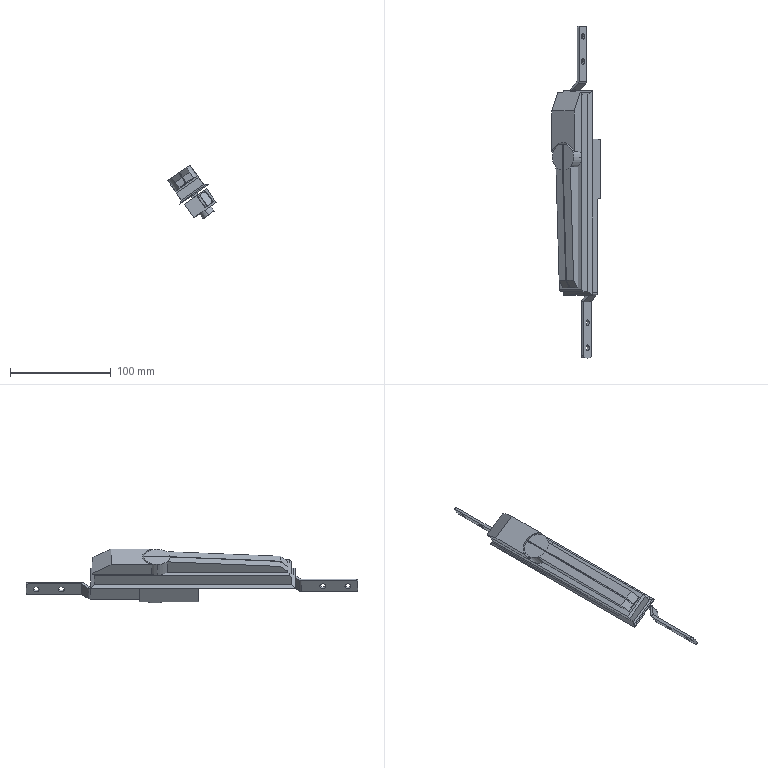Component | SolidWorks | MS830ConnectingRodLock-1 | 3 solids | 171 faces | volume 145170 mm3 | plane 130 | cylinder 41 | commonest cylinder face diameters 6 x8 26 x5 0.4 x4 5.4 x4 4 x4 13.5 x4 5 x4 7 x4